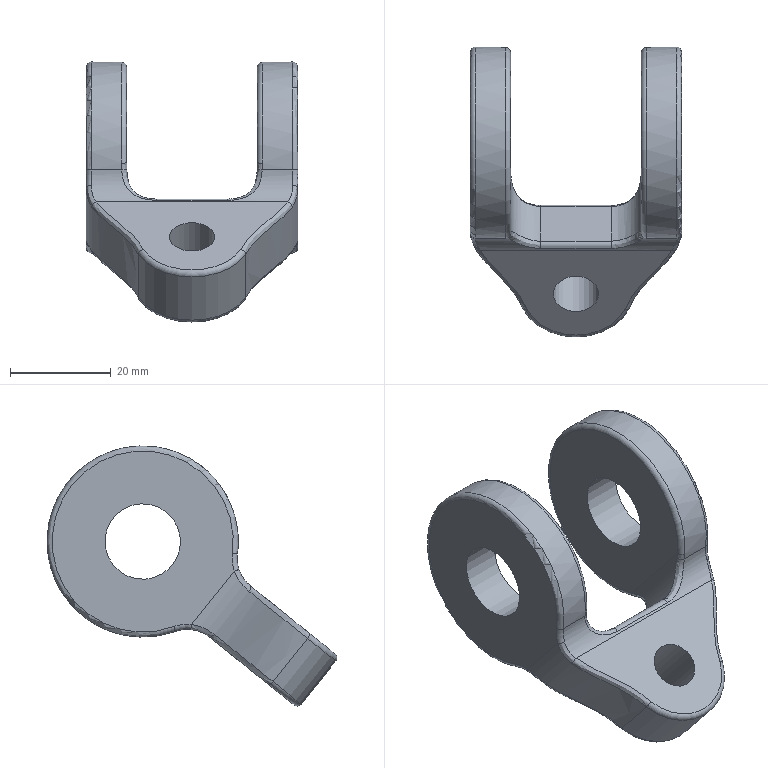CAM job | NX | mm | 3-axis | 3 set-ups | 8 operations | part box 42 x 57.59 x 51.7
set-up 1
1. Cavity Milling | Mill Mill5 D10 | CAVITY_MILL | path 126565.989 mm | 25.646 min
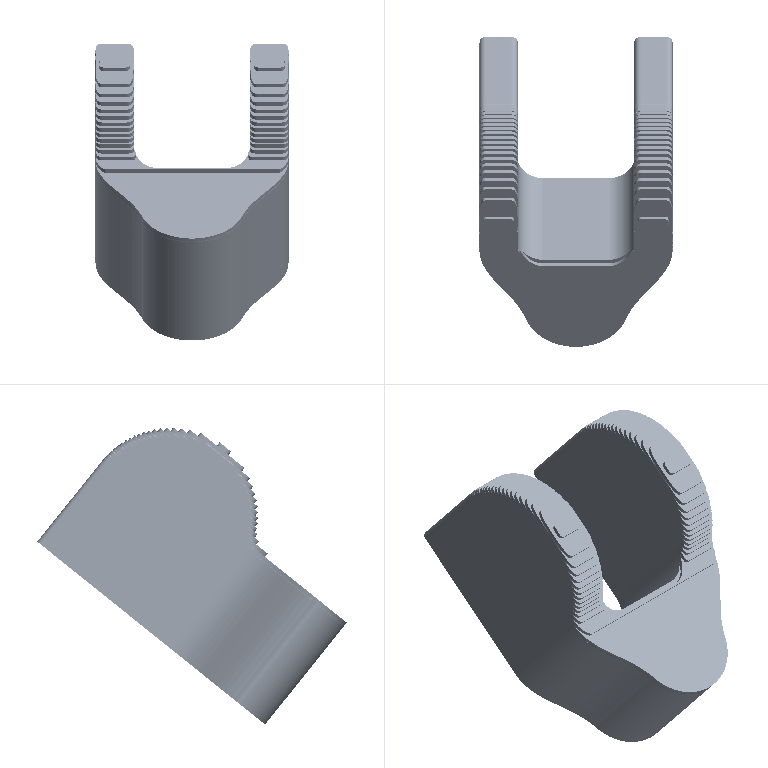2. Volume Based 2.5D Milling | Mill Mill5 D10 | FLOOR_WALL_COPY | path 261.759 mm | 0.2754 min
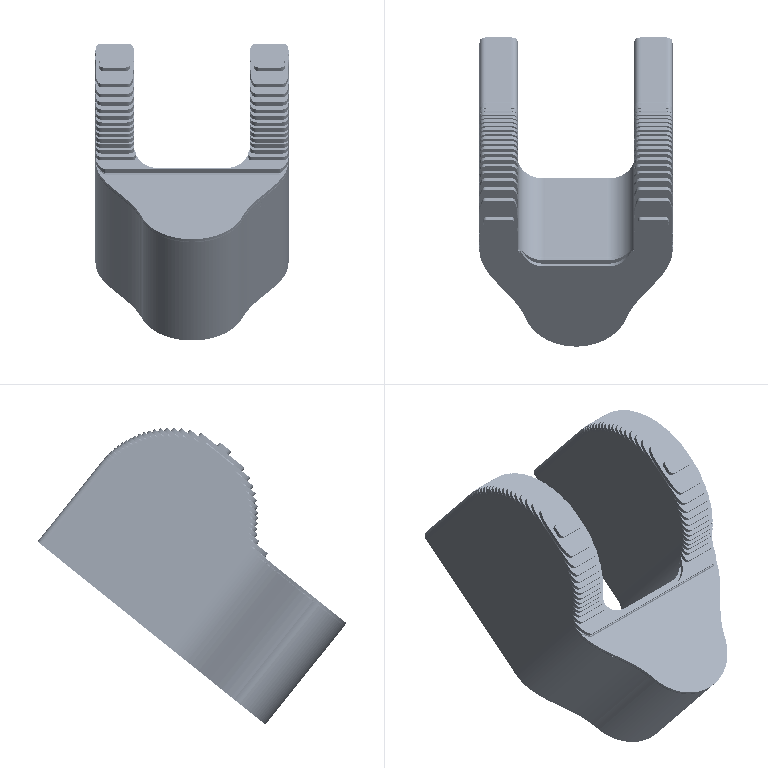3. Z-Level Milling | Mill Mill5 D10R5 | ZLEVEL_PROFILE | path 22559.13 mm | 18.252 min
4. Cylinder Milling | Mill Mill5 D6 | HOLE_MILLING | path 610.478 mm | 0.9203 min
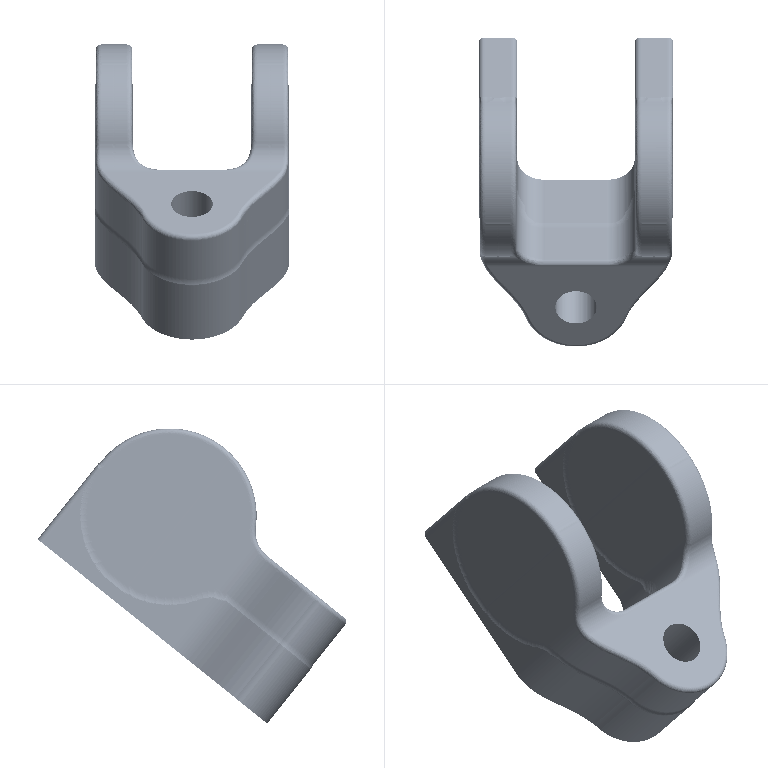set-up 2
5. Cavity Milling | Mill Mill5 D10 | CAVITY_MILL_COPY | path 20022.989 mm | 5.352 min
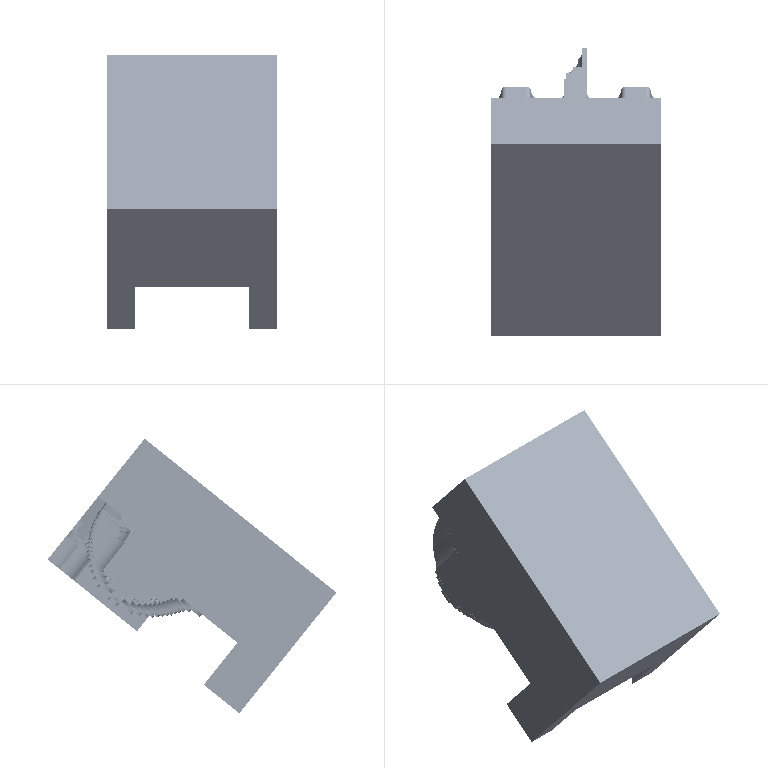6. Volume Based 2.5D Milling | Mill Mill5 D10 | FLOOR_WALL_COPY_COPY | path 261.758 mm | 0.2754 min
7. Fixed-axis Surface Contouring | Mill Mill5 D10R5 | FIXED_CONTOUR | path 6925.058 mm | 5.598 min
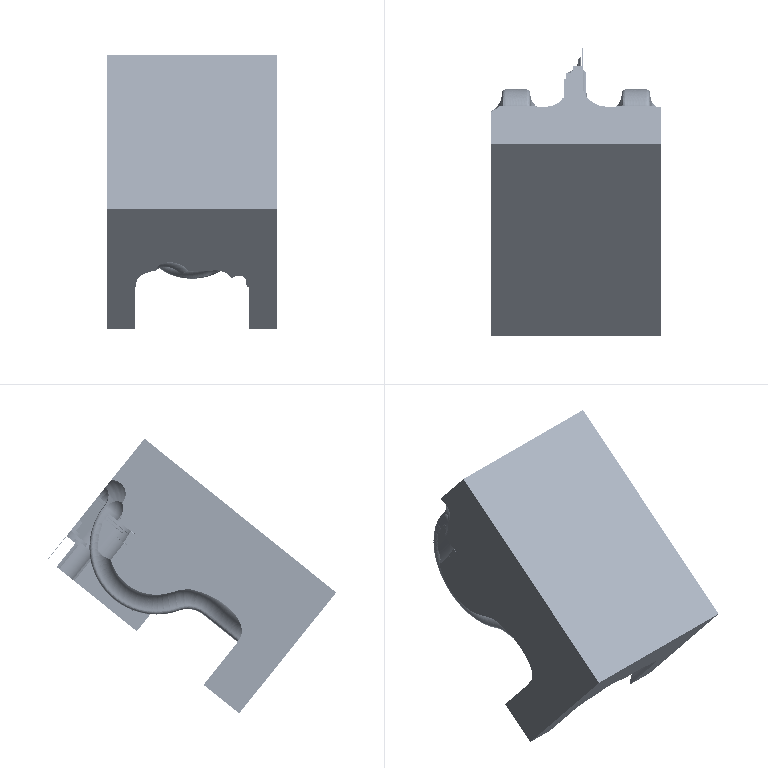set-up 3
8. Cylinder Milling | Mill Mill5 D10 | HOLE_MILLING_COPY | path 2498.556 mm | 4.061 min